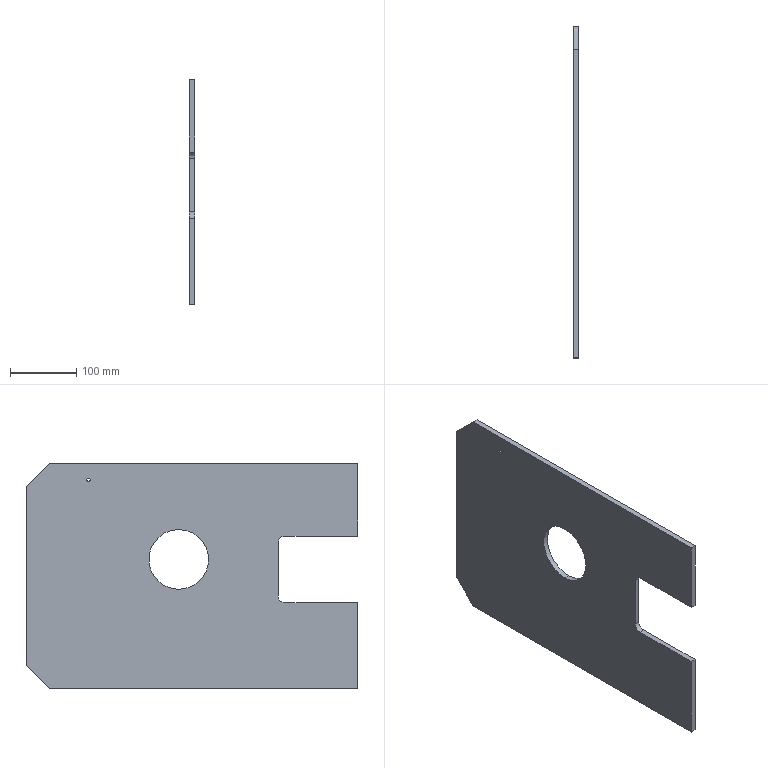Component | SolidWorks | THK-A1003LiftingSupportPlateRight-1 | 1 solid | 18 faces | box 8 x 500 x 340 mm | volume 1203492 mm3 | plane 12 | cylinder 6 | commonest cylinder face diameters 5 x2 90 x2 20 x2 | material Q235A
build123d program:
from build123d import *

# Parameters (mm, degrees)
SKETCH1_R           = 45
BOSS_EXTRUDE1_DEPTH = 4
CHAMFER1_SIZE       = 35
M6_TAPPED_HOLE1_D   = 5


with BuildPart() as part:
    # Sketch1 → Boss-Extrude1 (new, symmetric)
    with BuildSketch(Plane.ZY):
        with BuildLine():
            Line((-195, 230), (145, 230))
            Line((145, 230), (145, -270))
            Line((145, -270), (35, -270))
            Line((35, -270), (35, -160))
            ThreePointArc((35, -160), (32.071, -152.929), (25, -150))
            Line((25, -150), (-55, -150))
            ThreePointArc((-55, -150), (-62.071, -152.929), (-65, -160))
            Line((-65, -160), (-65, -270))
            Line((-65, -270), (-195, -270))
            Line((-195, -270), (-195, 230))
        make_face()
        Circle(SKETCH1_R, mode=Mode.SUBTRACT)
    extrude(amount=BOSS_EXTRUDE1_DEPTH, both=True)

    # Chamfer1
    chamfer1_edges = [part.edges().sort_by_distance(p)[0] for p in [
        (0, 230, -195),
        (0, 230, 145),
    ]]
    chamfer(chamfer1_edges, length=CHAMFER1_SIZE)

    # M6 Tapped Hole1 (through all)
    with Locations(Plane(origin=(4, 0, 0), x_dir=(0, 0, -1), z_dir=(1, 0, 0))):
        with Locations((-120, 136)):
            Hole(M6_TAPPED_HOLE1_D / 2)


solid = part.part

# Placed as in the assembly
solid = solid.moved(Location((120, 383, -155), (0, 0, 0)))
STEP:
#1=CARTESIAN_POINT('',(4.567,20.433,-1.28));
#2=VERTEX_POINT('',#1);
#3=CARTESIAN_POINT('',(4.567,20.433,-1.476));
#4=VERTEX_POINT('',#3);
#5=CARTESIAN_POINT('',(4.567,20.433,-1.378));
#6=DIRECTION('',(1.,0.,0.));
#7=DIRECTION('',(0.,0.,-1.));
#8=AXIS2_PLACEMENT_3D('',#5,#6,#7);
#9=CIRCLE('',#8,0.09843);
#10=EDGE_CURVE('',#2,#4,#9,.T.);
#11=ORIENTED_EDGE('',*,*,#10,.F.);
#12=CARTESIAN_POINT('',(4.882,20.433,-1.28));
#13=VERTEX_POINT('',#12);
#14=CARTESIAN_POINT('',(4.882,20.433,-1.28));
#15=DIRECTION('',(1.,0.,0.));
#16=VECTOR('',#15,39.37);
#17=LINE('',#14,#16);
#18=EDGE_CURVE('',#2,#13,#17,.T.);
#19=ORIENTED_EDGE('',*,*,#18,.T.);
#20=CARTESIAN_POINT('',(4.882,20.433,-1.476));
#21=VERTEX_POINT('',#20);
#22=CARTESIAN_POINT('',(4.882,20.433,-1.378));
#23=DIRECTION('',(1.,0.,0.));
#24=DIRECTION('',(0.,0.,-1.));
#25=AXIS2_PLACEMENT_3D('',#22,#23,#24);
#26=CIRCLE('',#25,0.09843);
#27=EDGE_CURVE('',#13,#21,#26,.T.);
#28=ORIENTED_EDGE('',*,*,#27,.T.);
#29=CARTESIAN_POINT('',(4.882,20.433,-1.476));
#30=DIRECTION('',(1.,0.,0.));
#31=VECTOR('',#30,39.37);
#32=LINE('',#29,#31);
#33=EDGE_CURVE('',#4,#21,#32,.T.);
#34=ORIENTED_EDGE('',*,*,#33,.F.);
#35=EDGE_LOOP('',(#11,#19,#28,#34));
#36=FACE_OUTER_BOUND('',#35,.T.);
#37=CARTESIAN_POINT('',(4.882,20.433,-1.378));
#38=DIRECTION('',(1.,0.,0.));
#39=DIRECTION('',(0.,0.,-1.));
#40=AXIS2_PLACEMENT_3D('',#37,#38,#39);
#41=CYLINDRICAL_SURFACE('',#40,0.09843);
#42=ADVANCED_FACE('',(#36),#41,.F.);
#43=CARTESIAN_POINT('',(4.567,15.079,-7.874));
#44=VERTEX_POINT('',#43);
#45=CARTESIAN_POINT('',(4.567,15.079,-4.331));
#46=VERTEX_POINT('',#45);
#47=CARTESIAN_POINT('',(4.567,15.079,-6.102));
#48=DIRECTION('',(-1.,0.,0.));
#49=DIRECTION('',(0.,0.,1.));
#50=AXIS2_PLACEMENT_3D('',#47,#48,#49);
#51=CIRCLE('',#50,1.772);
#52=EDGE_CURVE('',#44,#46,#51,.T.);
#53=ORIENTED_EDGE('',*,*,#52,.T.);
#54=CARTESIAN_POINT('',(4.882,15.079,-4.331));
#55=VERTEX_POINT('',#54);
#56=CARTESIAN_POINT('',(4.567,15.079,-4.331));
#57=DIRECTION('',(1.,0.,0.));
#58=VECTOR('',#57,39.37);
#59=LINE('',#56,#58);
#60=EDGE_CURVE('',#46,#55,#59,.T.);
#61=ORIENTED_EDGE('',*,*,#60,.T.);
#62=CARTESIAN_POINT('',(4.882,15.079,-7.874));
#63=VERTEX_POINT('',#62);
#64=CARTESIAN_POINT('',(4.882,15.079,-6.102));
#65=DIRECTION('',(-1.,0.,0.));
#66=DIRECTION('',(0.,0.,1.));
#67=AXIS2_PLACEMENT_3D('',#64,#65,#66);
#68=CIRCLE('',#67,1.772);
#69=EDGE_CURVE('',#63,#55,#68,.T.);
#70=ORIENTED_EDGE('',*,*,#69,.F.);
#71=CARTESIAN_POINT('',(4.567,15.079,-7.874));
#72=DIRECTION('',(1.,0.,0.));
#73=VECTOR('',#72,39.37);
#74=LINE('',#71,#73);
#75=EDGE_CURVE('',#44,#63,#74,.T.);
#76=ORIENTED_EDGE('',*,*,#75,.F.);
#77=EDGE_LOOP('',(#53,#61,#70,#76));
#78=FACE_OUTER_BOUND('',#77,.T.);
#79=CARTESIAN_POINT('',(4.567,15.079,-6.102));
#80=DIRECTION('',(1.,0.,0.));
#81=DIRECTION('',(0.,0.,-1.));
#82=AXIS2_PLACEMENT_3D('',#79,#80,#81);
#83=CYLINDRICAL_SURFACE('',#82,1.772);
#84=ADVANCED_FACE('',(#78),#83,.F.);
#85=CARTESIAN_POINT('',(4.567,20.433,-1.378));
#86=DIRECTION('',(1.,0.,0.));
#87=DIRECTION('',(0.,0.,-1.));
#88=AXIS2_PLACEMENT_3D('',#85,#86,#87);
#89=CIRCLE('',#88,0.09843);
#90=EDGE_CURVE('',#4,#2,#89,.T.);
#91=ORIENTED_EDGE('',*,*,#90,.T.);
#92=ORIENTED_EDGE('',*,*,#10,.T.);
#93=EDGE_LOOP('',(#91,#92));
#94=FACE_BOUND('',#93,.T.);
#95=CARTESIAN_POINT('',(4.567,24.134,-1.772));
#96=VERTEX_POINT('',#95);
#97=CARTESIAN_POINT('',(4.567,24.134,-12.402));
#98=VERTEX_POINT('',#97);
#99=CARTESIAN_POINT('',(4.567,24.134,-13.78));
#100=DIRECTION('',(0.,0.,-1.));
#101=VECTOR('',#100,39.37);
#102=LINE('',#99,#101);
#103=EDGE_CURVE('',#96,#98,#102,.T.);
#104=ORIENTED_EDGE('',*,*,#103,.T.);
#105=CARTESIAN_POINT('',(4.567,22.756,-13.78));
#106=VERTEX_POINT('',#105);
#107=CARTESIAN_POINT('',(4.567,20.098,-16.437));
#108=DIRECTION('',(0.,-0.7071,-0.7071));
#109=VECTOR('',#108,39.37);
#110=LINE('',#107,#109);
#111=EDGE_CURVE('',#98,#106,#110,.T.);
#112=ORIENTED_EDGE('',*,*,#111,.T.);
#113=CARTESIAN_POINT('',(4.567,4.449,-13.78));
#114=VERTEX_POINT('',#113);
#115=CARTESIAN_POINT('',(4.567,4.449,-13.78));
#116=DIRECTION('',(0.,-1.,0.));
#117=VECTOR('',#116,39.37);
#118=LINE('',#115,#117);
#119=EDGE_CURVE('',#106,#114,#118,.T.);
#120=ORIENTED_EDGE('',*,*,#119,.T.);
#121=CARTESIAN_POINT('',(4.567,4.449,-8.661));
#122=VERTEX_POINT('',#121);
#123=CARTESIAN_POINT('',(4.567,4.449,-8.661));
#124=DIRECTION('',(0.,0.,1.));
#125=VECTOR('',#124,39.37);
#126=LINE('',#123,#125);
#127=EDGE_CURVE('',#114,#122,#126,.T.);
#128=ORIENTED_EDGE('',*,*,#127,.T.);
#129=CARTESIAN_POINT('',(4.567,8.78,-8.661));
#130=VERTEX_POINT('',#129);
#131=CARTESIAN_POINT('',(4.567,8.78,-8.661));
#132=DIRECTION('',(0.,1.,-0.));
#133=VECTOR('',#132,39.37);
#134=LINE('',#131,#133);
#135=EDGE_CURVE('',#122,#130,#134,.T.);
#136=ORIENTED_EDGE('',*,*,#135,.T.);
#137=CARTESIAN_POINT('',(4.567,9.173,-8.268));
#138=VERTEX_POINT('',#137);
#139=CARTESIAN_POINT('',(4.567,8.78,-8.268));
#140=DIRECTION('',(1.,0.,0.));
#141=DIRECTION('',(0.,0.,-1.));
#142=AXIS2_PLACEMENT_3D('',#139,#140,#141);
#143=CIRCLE('',#142,0.3937);
#144=EDGE_CURVE('',#130,#138,#143,.T.);
#145=ORIENTED_EDGE('',*,*,#144,.T.);
#146=CARTESIAN_POINT('',(4.567,9.173,-5.118));
#147=VERTEX_POINT('',#146);
#148=CARTESIAN_POINT('',(4.567,9.173,-5.118));
#149=DIRECTION('',(0.,0.,1.));
#150=VECTOR('',#149,39.37);
#151=LINE('',#148,#150);
#152=EDGE_CURVE('',#138,#147,#151,.T.);
#153=ORIENTED_EDGE('',*,*,#152,.T.);
#154=CARTESIAN_POINT('',(4.567,8.78,-4.724));
#155=VERTEX_POINT('',#154);
#156=CARTESIAN_POINT('',(4.567,8.78,-5.118));
#157=DIRECTION('',(1.,0.,0.));
#158=DIRECTION('',(0.,0.,1.));
#159=AXIS2_PLACEMENT_3D('',#156,#157,#158);
#160=CIRCLE('',#159,0.3937);
#161=EDGE_CURVE('',#147,#155,#160,.T.);
#162=ORIENTED_EDGE('',*,*,#161,.T.);
#163=CARTESIAN_POINT('',(4.567,4.449,-4.724));
#164=VERTEX_POINT('',#163);
#165=CARTESIAN_POINT('',(4.567,4.449,-4.724));
#166=DIRECTION('',(0.,-1.,0.));
#167=VECTOR('',#166,39.37);
#168=LINE('',#165,#167);
#169=EDGE_CURVE('',#155,#164,#168,.T.);
#170=ORIENTED_EDGE('',*,*,#169,.T.);
#171=CARTESIAN_POINT('',(4.567,4.449,-0.3937));
#172=VERTEX_POINT('',#171);
#173=CARTESIAN_POINT('',(4.567,4.449,-0.3937));
#174=DIRECTION('',(0.,0.,1.));
#175=VECTOR('',#174,39.37);
#176=LINE('',#173,#175);
#177=EDGE_CURVE('',#164,#172,#176,.T.);
#178=ORIENTED_EDGE('',*,*,#177,.T.);
#179=CARTESIAN_POINT('',(4.567,22.756,-0.3937));
#180=VERTEX_POINT('',#179);
#181=CARTESIAN_POINT('',(4.567,24.134,-0.3937));
#182=DIRECTION('',(0.,1.,-0.));
#183=VECTOR('',#182,39.37);
#184=LINE('',#181,#183);
#185=EDGE_CURVE('',#172,#180,#184,.T.);
#186=ORIENTED_EDGE('',*,*,#185,.T.);
#187=CARTESIAN_POINT('',(4.567,18.13,4.232));
#188=DIRECTION('',(0.,0.7071,-0.7071));
#189=VECTOR('',#188,39.37);
#190=LINE('',#187,#189);
#191=EDGE_CURVE('',#180,#96,#190,.T.);
#192=ORIENTED_EDGE('',*,*,#191,.T.);
#193=EDGE_LOOP('',(#104,#112,#120,#128,#136,#145,#153,#162,#170,#178,#186,#192));
#194=FACE_OUTER_BOUND('',#193,.T.);
#195=ORIENTED_EDGE('',*,*,#52,.F.);
#196=CARTESIAN_POINT('',(4.567,15.079,-6.102));
#197=DIRECTION('',(-1.,0.,0.));
#198=DIRECTION('',(0.,0.,1.));
#199=AXIS2_PLACEMENT_3D('',#196,#197,#198);
#200=CIRCLE('',#199,1.772);
#201=EDGE_CURVE('',#46,#44,#200,.T.);
#202=ORIENTED_EDGE('',*,*,#201,.F.);
#203=EDGE_LOOP('',(#195,#202));
#204=FACE_BOUND('',#203,.T.);
#205=CARTESIAN_POINT('',(4.567,8.78,-5.118));
#206=DIRECTION('',(-1.,0.,0.));
#207=DIRECTION('',(0.,0.,1.));
#208=AXIS2_PLACEMENT_3D('',#205,#206,#207);
#209=PLANE('',#208);
#210=ADVANCED_FACE('',(#94,#194,#204),#209,.T.);
#211=CARTESIAN_POINT('',(4.882,20.433,-1.378));
#212=DIRECTION('',(1.,0.,0.));
#213=DIRECTION('',(0.,0.,-1.));
#214=AXIS2_PLACEMENT_3D('',#211,#212,#213);
#215=CIRCLE('',#214,0.09843);
#216=EDGE_CURVE('',#21,#13,#215,.T.);
#217=ORIENTED_EDGE('',*,*,#216,.F.);
#218=ORIENTED_EDGE('',*,*,#27,.F.);
#219=EDGE_LOOP('',(#217,#218));
#220=FACE_BOUND('',#219,.T.);
#221=CARTESIAN_POINT('',(4.882,22.756,-13.78));
#222=VERTEX_POINT('',#221);
#223=CARTESIAN_POINT('',(4.882,4.449,-13.78));
#224=VERTEX_POINT('',#223);
#225=CARTESIAN_POINT('',(4.882,4.449,-13.78));
#226=DIRECTION('',(0.,-1.,0.));
#227=VECTOR('',#226,39.37);
#228=LINE('',#225,#227);
#229=EDGE_CURVE('',#222,#224,#228,.T.);
#230=ORIENTED_EDGE('',*,*,#229,.F.);
#231=CARTESIAN_POINT('',(4.882,24.134,-12.402));
#232=VERTEX_POINT('',#231);
#233=CARTESIAN_POINT('',(4.882,22.756,-13.78));
#234=DIRECTION('',(0.,0.7071,0.7071));
#235=VECTOR('',#234,39.37);
#236=LINE('',#233,#235);
#237=EDGE_CURVE('',#222,#232,#236,.T.);
#238=ORIENTED_EDGE('',*,*,#237,.T.);
#239=CARTESIAN_POINT('',(4.882,24.134,-1.772));
#240=VERTEX_POINT('',#239);
#241=CARTESIAN_POINT('',(4.882,24.134,-13.78));
#242=DIRECTION('',(0.,0.,-1.));
#243=VECTOR('',#242,39.37);
#244=LINE('',#241,#243);
#245=EDGE_CURVE('',#240,#232,#244,.T.);
#246=ORIENTED_EDGE('',*,*,#245,.F.);
#247=CARTESIAN_POINT('',(4.882,22.756,-0.3937));
#248=VERTEX_POINT('',#247);
#249=CARTESIAN_POINT('',(4.882,24.134,-1.772));
#250=DIRECTION('',(0.,-0.7071,0.7071));
#251=VECTOR('',#250,39.37);
#252=LINE('',#249,#251);
#253=EDGE_CURVE('',#240,#248,#252,.T.);
#254=ORIENTED_EDGE('',*,*,#253,.T.);
#255=CARTESIAN_POINT('',(4.882,4.449,-0.3937));
#256=VERTEX_POINT('',#255);
#257=CARTESIAN_POINT('',(4.882,24.134,-0.3937));
#258=DIRECTION('',(0.,1.,-0.));
#259=VECTOR('',#258,39.37);
#260=LINE('',#257,#259);
#261=EDGE_CURVE('',#256,#248,#260,.T.);
#262=ORIENTED_EDGE('',*,*,#261,.F.);
#263=CARTESIAN_POINT('',(4.882,4.449,-4.724));
#264=VERTEX_POINT('',#263);
#265=CARTESIAN_POINT('',(4.882,4.449,-0.3937));
#266=DIRECTION('',(0.,0.,1.));
#267=VECTOR('',#266,39.37);
#268=LINE('',#265,#267);
#269=EDGE_CURVE('',#264,#256,#268,.T.);
#270=ORIENTED_EDGE('',*,*,#269,.F.);
#271=CARTESIAN_POINT('',(4.882,8.78,-4.724));
#272=VERTEX_POINT('',#271);
#273=CARTESIAN_POINT('',(4.882,4.449,-4.724));
#274=DIRECTION('',(0.,-1.,0.));
#275=VECTOR('',#274,39.37);
#276=LINE('',#273,#275);
#277=EDGE_CURVE('',#272,#264,#276,.T.);
#278=ORIENTED_EDGE('',*,*,#277,.F.);
#279=CARTESIAN_POINT('',(4.882,9.173,-5.118));
#280=VERTEX_POINT('',#279);
#281=CARTESIAN_POINT('',(4.882,8.78,-5.118));
#282=DIRECTION('',(1.,0.,0.));
#283=DIRECTION('',(0.,0.,1.));
#284=AXIS2_PLACEMENT_3D('',#281,#282,#283);
#285=CIRCLE('',#284,0.3937);
#286=EDGE_CURVE('',#280,#272,#285,.T.);
#287=ORIENTED_EDGE('',*,*,#286,.F.);
#288=CARTESIAN_POINT('',(4.882,9.173,-8.268));
#289=VERTEX_POINT('',#288);
#290=CARTESIAN_POINT('',(4.882,9.173,-5.118));
#291=DIRECTION('',(0.,0.,1.));
#292=VECTOR('',#291,39.37);
#293=LINE('',#290,#292);
#294=EDGE_CURVE('',#289,#280,#293,.T.);
#295=ORIENTED_EDGE('',*,*,#294,.F.);
#296=CARTESIAN_POINT('',(4.882,8.78,-8.661));
#297=VERTEX_POINT('',#296);
#298=CARTESIAN_POINT('',(4.882,8.78,-8.268));
#299=DIRECTION('',(1.,0.,0.));
#300=DIRECTION('',(0.,0.,-1.));
#301=AXIS2_PLACEMENT_3D('',#298,#299,#300);
#302=CIRCLE('',#301,0.3937);
#303=EDGE_CURVE('',#297,#289,#302,.T.);
#304=ORIENTED_EDGE('',*,*,#303,.F.);
#305=CARTESIAN_POINT('',(4.882,4.449,-8.661));
#306=VERTEX_POINT('',#305);
#307=CARTESIAN_POINT('',(4.882,8.78,-8.661));
#308=DIRECTION('',(0.,1.,-0.));
#309=VECTOR('',#308,39.37);
#310=LINE('',#307,#309);
#311=EDGE_CURVE('',#306,#297,#310,.T.);
#312=ORIENTED_EDGE('',*,*,#311,.F.);
#313=CARTESIAN_POINT('',(4.882,4.449,-8.661));
#314=DIRECTION('',(0.,0.,1.));
#315=VECTOR('',#314,39.37);
#316=LINE('',#313,#315);
#317=EDGE_CURVE('',#224,#306,#316,.T.);
#318=ORIENTED_EDGE('',*,*,#317,.F.);
#319=EDGE_LOOP('',(#230,#238,#246,#254,#262,#270,#278,#287,#295,#304,#312,#318));
#320=FACE_OUTER_BOUND('',#319,.T.);
#321=ORIENTED_EDGE('',*,*,#69,.T.);
#322=CARTESIAN_POINT('',(4.882,15.079,-6.102));
#323=DIRECTION('',(-1.,0.,0.));
#324=DIRECTION('',(0.,0.,1.));
#325=AXIS2_PLACEMENT_3D('',#322,#323,#324);
#326=CIRCLE('',#325,1.772);
#327=EDGE_CURVE('',#55,#63,#326,.T.);
#328=ORIENTED_EDGE('',*,*,#327,.T.);
#329=EDGE_LOOP('',(#321,#328));
#330=FACE_BOUND('',#329,.T.);
#331=CARTESIAN_POINT('',(4.882,8.78,-5.118));
#332=DIRECTION('',(-1.,0.,0.));
#333=DIRECTION('',(0.,0.,1.));
#334=AXIS2_PLACEMENT_3D('',#331,#332,#333);
#335=PLANE('',#334);
#336=ADVANCED_FACE('',(#220,#320,#330),#335,.F.);
#337=ORIENTED_EDGE('',*,*,#119,.F.);
#338=CARTESIAN_POINT('',(4.567,22.756,-13.78));
#339=DIRECTION('',(1.,0.,0.));
#340=VECTOR('',#339,39.37);
#341=LINE('',#338,#340);
#342=EDGE_CURVE('',#106,#222,#341,.T.);
#343=ORIENTED_EDGE('',*,*,#342,.T.);
#344=ORIENTED_EDGE('',*,*,#229,.T.);
#345=CARTESIAN_POINT('',(4.567,4.449,-13.78));
#346=DIRECTION('',(1.,0.,0.));
#347=VECTOR('',#346,39.37);
#348=LINE('',#345,#347);
#349=EDGE_CURVE('',#114,#224,#348,.T.);
#350=ORIENTED_EDGE('',*,*,#349,.F.);
#351=EDGE_LOOP('',(#337,#343,#344,#350));
#352=FACE_OUTER_BOUND('',#351,.T.);
#353=CARTESIAN_POINT('',(4.567,4.449,-13.78));
#354=DIRECTION('',(0.,0.,1.));
#355=DIRECTION('',(1.,0.,0.));
#356=AXIS2_PLACEMENT_3D('',#353,#354,#355);
#357=PLANE('',#356);
#358=ADVANCED_FACE('',(#352),#357,.F.);
#359=ORIENTED_EDGE('',*,*,#317,.T.);
#360=CARTESIAN_POINT('',(4.567,4.449,-8.661));
#361=DIRECTION('',(1.,0.,0.));
#362=VECTOR('',#361,39.37);
#363=LINE('',#360,#362);
#364=EDGE_CURVE('',#122,#306,#363,.T.);
#365=ORIENTED_EDGE('',*,*,#364,.F.);
#366=ORIENTED_EDGE('',*,*,#127,.F.);
#367=ORIENTED_EDGE('',*,*,#349,.T.);
#368=EDGE_LOOP('',(#359,#365,#366,#367));
#369=FACE_OUTER_BOUND('',#368,.T.);
#370=CARTESIAN_POINT('',(4.567,4.449,-8.661));
#371=DIRECTION('',(0.,1.,0.));
#372=DIRECTION('',(0.,0.,1.));
#373=AXIS2_PLACEMENT_3D('',#370,#371,#372);
#374=PLANE('',#373);
#375=ADVANCED_FACE('',(#369),#374,.F.);
#376=ORIENTED_EDGE('',*,*,#311,.T.);
#377=CARTESIAN_POINT('',(4.567,8.78,-8.661));
#378=DIRECTION('',(1.,0.,0.));
#379=VECTOR('',#378,39.37);
#380=LINE('',#377,#379);
#381=EDGE_CURVE('',#130,#297,#380,.T.);
#382=ORIENTED_EDGE('',*,*,#381,.F.);
#383=ORIENTED_EDGE('',*,*,#135,.F.);
#384=ORIENTED_EDGE('',*,*,#364,.T.);
#385=EDGE_LOOP('',(#376,#382,#383,#384));
#386=FACE_OUTER_BOUND('',#385,.T.);
#387=CARTESIAN_POINT('',(4.567,8.78,-8.661));
#388=DIRECTION('',(0.,-0.,-1.));
#389=DIRECTION('',(0.,1.,-0.));
#390=AXIS2_PLACEMENT_3D('',#387,#388,#389);
#391=PLANE('',#390);
#392=ADVANCED_FACE('',(#386),#391,.F.);
#393=ORIENTED_EDGE('',*,*,#303,.T.);
#394=CARTESIAN_POINT('',(4.567,9.173,-8.268));
#395=DIRECTION('',(1.,0.,0.));
#396=VECTOR('',#395,39.37);
#397=LINE('',#394,#396);
#398=EDGE_CURVE('',#138,#289,#397,.T.);
#399=ORIENTED_EDGE('',*,*,#398,.F.);
#400=ORIENTED_EDGE('',*,*,#144,.F.);
#401=ORIENTED_EDGE('',*,*,#381,.T.);
#402=EDGE_LOOP('',(#393,#399,#400,#401));
#403=FACE_OUTER_BOUND('',#402,.T.);
#404=CARTESIAN_POINT('',(4.567,8.78,-8.268));
#405=DIRECTION('',(1.,0.,0.));
#406=DIRECTION('',(0.,0.,-1.));
#407=AXIS2_PLACEMENT_3D('',#404,#405,#406);
#408=CYLINDRICAL_SURFACE('',#407,0.3937);
#409=ADVANCED_FACE('',(#403),#408,.F.);
#410=ORIENTED_EDGE('',*,*,#294,.T.);
#411=CARTESIAN_POINT('',(4.567,9.173,-5.118));
#412=DIRECTION('',(1.,0.,0.));
#413=VECTOR('',#412,39.37);
#414=LINE('',#411,#413);
#415=EDGE_CURVE('',#147,#280,#414,.T.);
#416=ORIENTED_EDGE('',*,*,#415,.F.);
#417=ORIENTED_EDGE('',*,*,#152,.F.);
#418=ORIENTED_EDGE('',*,*,#398,.T.);
#419=EDGE_LOOP('',(#410,#416,#417,#418));
#420=FACE_OUTER_BOUND('',#419,.T.);
#421=CARTESIAN_POINT('',(4.567,9.173,-5.118));
#422=DIRECTION('',(0.,1.,0.));
#423=DIRECTION('',(0.,0.,1.));
#424=AXIS2_PLACEMENT_3D('',#421,#422,#423);
#425=PLANE('',#424);
#426=ADVANCED_FACE('',(#420),#425,.F.);
#427=ORIENTED_EDGE('',*,*,#286,.T.);
#428=CARTESIAN_POINT('',(4.567,8.78,-4.724));
#429=DIRECTION('',(1.,0.,0.));
#430=VECTOR('',#429,39.37);
#431=LINE('',#428,#430);
#432=EDGE_CURVE('',#155,#272,#431,.T.);
#433=ORIENTED_EDGE('',*,*,#432,.F.);
#434=ORIENTED_EDGE('',*,*,#161,.F.);
#435=ORIENTED_EDGE('',*,*,#415,.T.);
#436=EDGE_LOOP('',(#427,#433,#434,#435));
#437=FACE_OUTER_BOUND('',#436,.T.);
#438=CARTESIAN_POINT('',(4.567,8.78,-5.118));
#439=DIRECTION('',(1.,0.,0.));
#440=DIRECTION('',(0.,0.,-1.));
#441=AXIS2_PLACEMENT_3D('',#438,#439,#440);
#442=CYLINDRICAL_SURFACE('',#441,0.3937);
#443=ADVANCED_FACE('',(#437),#442,.F.);
#444=ORIENTED_EDGE('',*,*,#277,.T.);
#445=CARTESIAN_POINT('',(4.567,4.449,-4.724));
#446=DIRECTION('',(1.,0.,0.));
#447=VECTOR('',#446,39.37);
#448=LINE('',#445,#447);
#449=EDGE_CURVE('',#164,#264,#448,.T.);
#450=ORIENTED_EDGE('',*,*,#449,.F.);
#451=ORIENTED_EDGE('',*,*,#169,.F.);
#452=ORIENTED_EDGE('',*,*,#432,.T.);
#453=EDGE_LOOP('',(#444,#450,#451,#452));
#454=FACE_OUTER_BOUND('',#453,.T.);
#455=CARTESIAN_POINT('',(4.567,4.449,-4.724));
#456=DIRECTION('',(0.,0.,1.));
#457=DIRECTION('',(0.,-1.,0.));
#458=AXIS2_PLACEMENT_3D('',#455,#456,#457);
#459=PLANE('',#458);
#460=ADVANCED_FACE('',(#454),#459,.F.);
#461=ORIENTED_EDGE('',*,*,#269,.T.);
#462=CARTESIAN_POINT('',(4.567,4.449,-0.3937));
#463=DIRECTION('',(1.,0.,0.));
#464=VECTOR('',#463,39.37);
#465=LINE('',#462,#464);
#466=EDGE_CURVE('',#172,#256,#465,.T.);
#467=ORIENTED_EDGE('',*,*,#466,.F.);
#468=ORIENTED_EDGE('',*,*,#177,.F.);
#469=ORIENTED_EDGE('',*,*,#449,.T.);
#470=EDGE_LOOP('',(#461,#467,#468,#469));
#471=FACE_OUTER_BOUND('',#470,.T.);
#472=CARTESIAN_POINT('',(4.567,4.449,-0.3937));
#473=DIRECTION('',(0.,1.,0.));
#474=DIRECTION('',(0.,0.,1.));
#475=AXIS2_PLACEMENT_3D('',#472,#473,#474);
#476=PLANE('',#475);
#477=ADVANCED_FACE('',(#471),#476,.F.);
#478=ORIENTED_EDGE('',*,*,#261,.T.);
#479=CARTESIAN_POINT('',(4.567,22.756,-0.3937));
#480=DIRECTION('',(-1.,0.,0.));
#481=VECTOR('',#480,39.37);
#482=LINE('',#479,#481);
#483=EDGE_CURVE('',#248,#180,#482,.T.);
#484=ORIENTED_EDGE('',*,*,#483,.T.);
#485=ORIENTED_EDGE('',*,*,#185,.F.);
#486=ORIENTED_EDGE('',*,*,#466,.T.);
#487=EDGE_LOOP('',(#478,#484,#485,#486));
#488=FACE_OUTER_BOUND('',#487,.T.);
#489=CARTESIAN_POINT('',(4.567,24.134,-0.3937));
#490=DIRECTION('',(0.,-0.,-1.));
#491=DIRECTION('',(0.,1.,-0.));
#492=AXIS2_PLACEMENT_3D('',#489,#490,#491);
#493=PLANE('',#492);
#494=ADVANCED_FACE('',(#488),#493,.F.);
#495=ORIENTED_EDGE('',*,*,#245,.T.);
#496=CARTESIAN_POINT('',(4.567,24.134,-12.402));
#497=DIRECTION('',(-1.,0.,0.));
#498=VECTOR('',#497,39.37);
#499=LINE('',#496,#498);
#500=EDGE_CURVE('',#232,#98,#499,.T.);
#501=ORIENTED_EDGE('',*,*,#500,.T.);
#502=ORIENTED_EDGE('',*,*,#103,.F.);
#503=CARTESIAN_POINT('',(4.567,24.134,-1.772));
#504=DIRECTION('',(1.,0.,0.));
#505=VECTOR('',#504,39.37);
#506=LINE('',#503,#505);
#507=EDGE_CURVE('',#96,#240,#506,.T.);
#508=ORIENTED_EDGE('',*,*,#507,.T.);
#509=EDGE_LOOP('',(#495,#501,#502,#508));
#510=FACE_OUTER_BOUND('',#509,.T.);
#511=CARTESIAN_POINT('',(4.567,24.134,-13.78));
#512=DIRECTION('',(0.,-1.,0.));
#513=DIRECTION('',(0.,0.,-1.));
#514=AXIS2_PLACEMENT_3D('',#511,#512,#513);
#515=PLANE('',#514);
#516=ADVANCED_FACE('',(#510),#515,.F.);
#517=ORIENTED_EDGE('',*,*,#60,.F.);
#518=ORIENTED_EDGE('',*,*,#201,.T.);
#519=ORIENTED_EDGE('',*,*,#75,.T.);
#520=ORIENTED_EDGE('',*,*,#327,.F.);
#521=EDGE_LOOP('',(#517,#518,#519,#520));
#522=FACE_OUTER_BOUND('',#521,.T.);
#523=CARTESIAN_POINT('',(4.567,15.079,-6.102));
#524=DIRECTION('',(1.,0.,0.));
#525=DIRECTION('',(0.,0.,-1.));
#526=AXIS2_PLACEMENT_3D('',#523,#524,#525);
#527=CYLINDRICAL_SURFACE('',#526,1.772);
#528=ADVANCED_FACE('',(#522),#527,.F.);
#529=ORIENTED_EDGE('',*,*,#111,.F.);
#530=ORIENTED_EDGE('',*,*,#500,.F.);
#531=ORIENTED_EDGE('',*,*,#237,.F.);
#532=ORIENTED_EDGE('',*,*,#342,.F.);
#533=EDGE_LOOP('',(#529,#530,#531,#532));
#534=FACE_OUTER_BOUND('',#533,.T.);
#535=CARTESIAN_POINT('',(4.567,22.756,-13.78));
#536=DIRECTION('',(0.,-0.7071,0.7071));
#537=DIRECTION('',(1.,0.,0.));
#538=AXIS2_PLACEMENT_3D('',#535,#536,#537);
#539=PLANE('',#538);
#540=ADVANCED_FACE('',(#534),#539,.F.);
#541=ORIENTED_EDGE('',*,*,#191,.F.);
#542=ORIENTED_EDGE('',*,*,#483,.F.);
#543=ORIENTED_EDGE('',*,*,#253,.F.);
#544=ORIENTED_EDGE('',*,*,#507,.F.);
#545=EDGE_LOOP('',(#541,#542,#543,#544));
#546=FACE_OUTER_BOUND('',#545,.T.);
#547=CARTESIAN_POINT('',(4.567,24.134,-1.772));
#548=DIRECTION('',(0.,-0.7071,-0.7071));
#549=DIRECTION('',(1.,0.,0.));
#550=AXIS2_PLACEMENT_3D('',#547,#548,#549);
#551=PLANE('',#550);
#552=ADVANCED_FACE('',(#546),#551,.F.);
#553=ORIENTED_EDGE('',*,*,#18,.F.);
#554=ORIENTED_EDGE('',*,*,#90,.F.);
#555=ORIENTED_EDGE('',*,*,#33,.T.);
#556=ORIENTED_EDGE('',*,*,#216,.T.);
#557=EDGE_LOOP('',(#553,#554,#555,#556));
#558=FACE_OUTER_BOUND('',#557,.T.);
#559=CARTESIAN_POINT('',(4.882,20.433,-1.378));
#560=DIRECTION('',(1.,0.,0.));
#561=DIRECTION('',(0.,0.,-1.));
#562=AXIS2_PLACEMENT_3D('',#559,#560,#561);
#563=CYLINDRICAL_SURFACE('',#562,0.09843);
#564=ADVANCED_FACE('',(#558),#563,.F.);
#565=CLOSED_SHELL('',(#42,#84,#210,#336,#358,#375,#392,#409,#426,#443,#460,#477,#494,#516,#528,#540,#552,#564));
#566=MANIFOLD_SOLID_BREP('',#565);
#567=CARTESIAN_POINT('',(0.,0.,0.));
#568=DIRECTION('',(0.,0.,1.));
#569=DIRECTION('',(1.,0.,0.));
#570=AXIS2_PLACEMENT_3D('',#567,#568,#569);
#571=(LENGTH_UNIT()NAMED_UNIT(*)SI_UNIT($,.METRE.));
#572=LENGTH_MEASURE_WITH_UNIT(LENGTH_MEASURE(0.0254),#571);
#573=DIMENSIONAL_EXPONENTS(1.,0.,0.,0.,0.,0.,0.);
#574=(CONVERSION_BASED_UNIT('',#572)LENGTH_UNIT()NAMED_UNIT(#573));
#575=UNCERTAINTY_MEASURE_WITH_UNIT(LENGTH_MEASURE(0.00001),#574,'','');
#576=(NAMED_UNIT(*)PLANE_ANGLE_UNIT()SI_UNIT($,.RADIAN.));
#577=(NAMED_UNIT(*)SI_UNIT($,.STERADIAN.)SOLID_ANGLE_UNIT());
#578=(GEOMETRIC_REPRESENTATION_CONTEXT(3)GLOBAL_UNCERTAINTY_ASSIGNED_CONTEXT((#575))GLOBAL_UNIT_ASSIGNED_CONTEXT((#574,#576,#577))REPRESENTATION_CONTEXT('',''));
#579=ADVANCED_BREP_SHAPE_REPRESENTATION('',(#566,#570),#578);
#580=COLOUR_RGB('',0.7922,0.8196,0.9333);
#581=FILL_AREA_STYLE_COLOUR('',#580);
#582=FILL_AREA_STYLE('',(#581));
#583=SURFACE_STYLE_FILL_AREA(#582);
#584=SURFACE_SIDE_STYLE('',(#583));
#585=SURFACE_STYLE_USAGE(.BOTH.,#584);
#586=PRESENTATION_STYLE_ASSIGNMENT((#585));
#587=STYLED_ITEM('',(#586),#566);
#588=(LENGTH_UNIT()NAMED_UNIT(*)SI_UNIT($,.METRE.));
#589=LENGTH_MEASURE_WITH_UNIT(LENGTH_MEASURE(0.0254),#588);
#590=DIMENSIONAL_EXPONENTS(1.,0.,0.,0.,0.,0.,0.);
#591=(CONVERSION_BASED_UNIT('',#589)LENGTH_UNIT()NAMED_UNIT(#590));
#592=UNCERTAINTY_MEASURE_WITH_UNIT(LENGTH_MEASURE(0.00001),#591,'','');
#593=(NAMED_UNIT(*)PLANE_ANGLE_UNIT()SI_UNIT($,.RADIAN.));
#594=(NAMED_UNIT(*)SI_UNIT($,.STERADIAN.)SOLID_ANGLE_UNIT());
#595=(GEOMETRIC_REPRESENTATION_CONTEXT(3)GLOBAL_UNCERTAINTY_ASSIGNED_CONTEXT((#592))GLOBAL_UNIT_ASSIGNED_CONTEXT((#591,#593,#594))REPRESENTATION_CONTEXT('',''));
#596=MECHANICAL_DESIGN_GEOMETRIC_PRESENTATION_REPRESENTATION('',(#587),#595);
#597=PRESENTATION_LAYER_ASSIGNMENT('','',(#587));